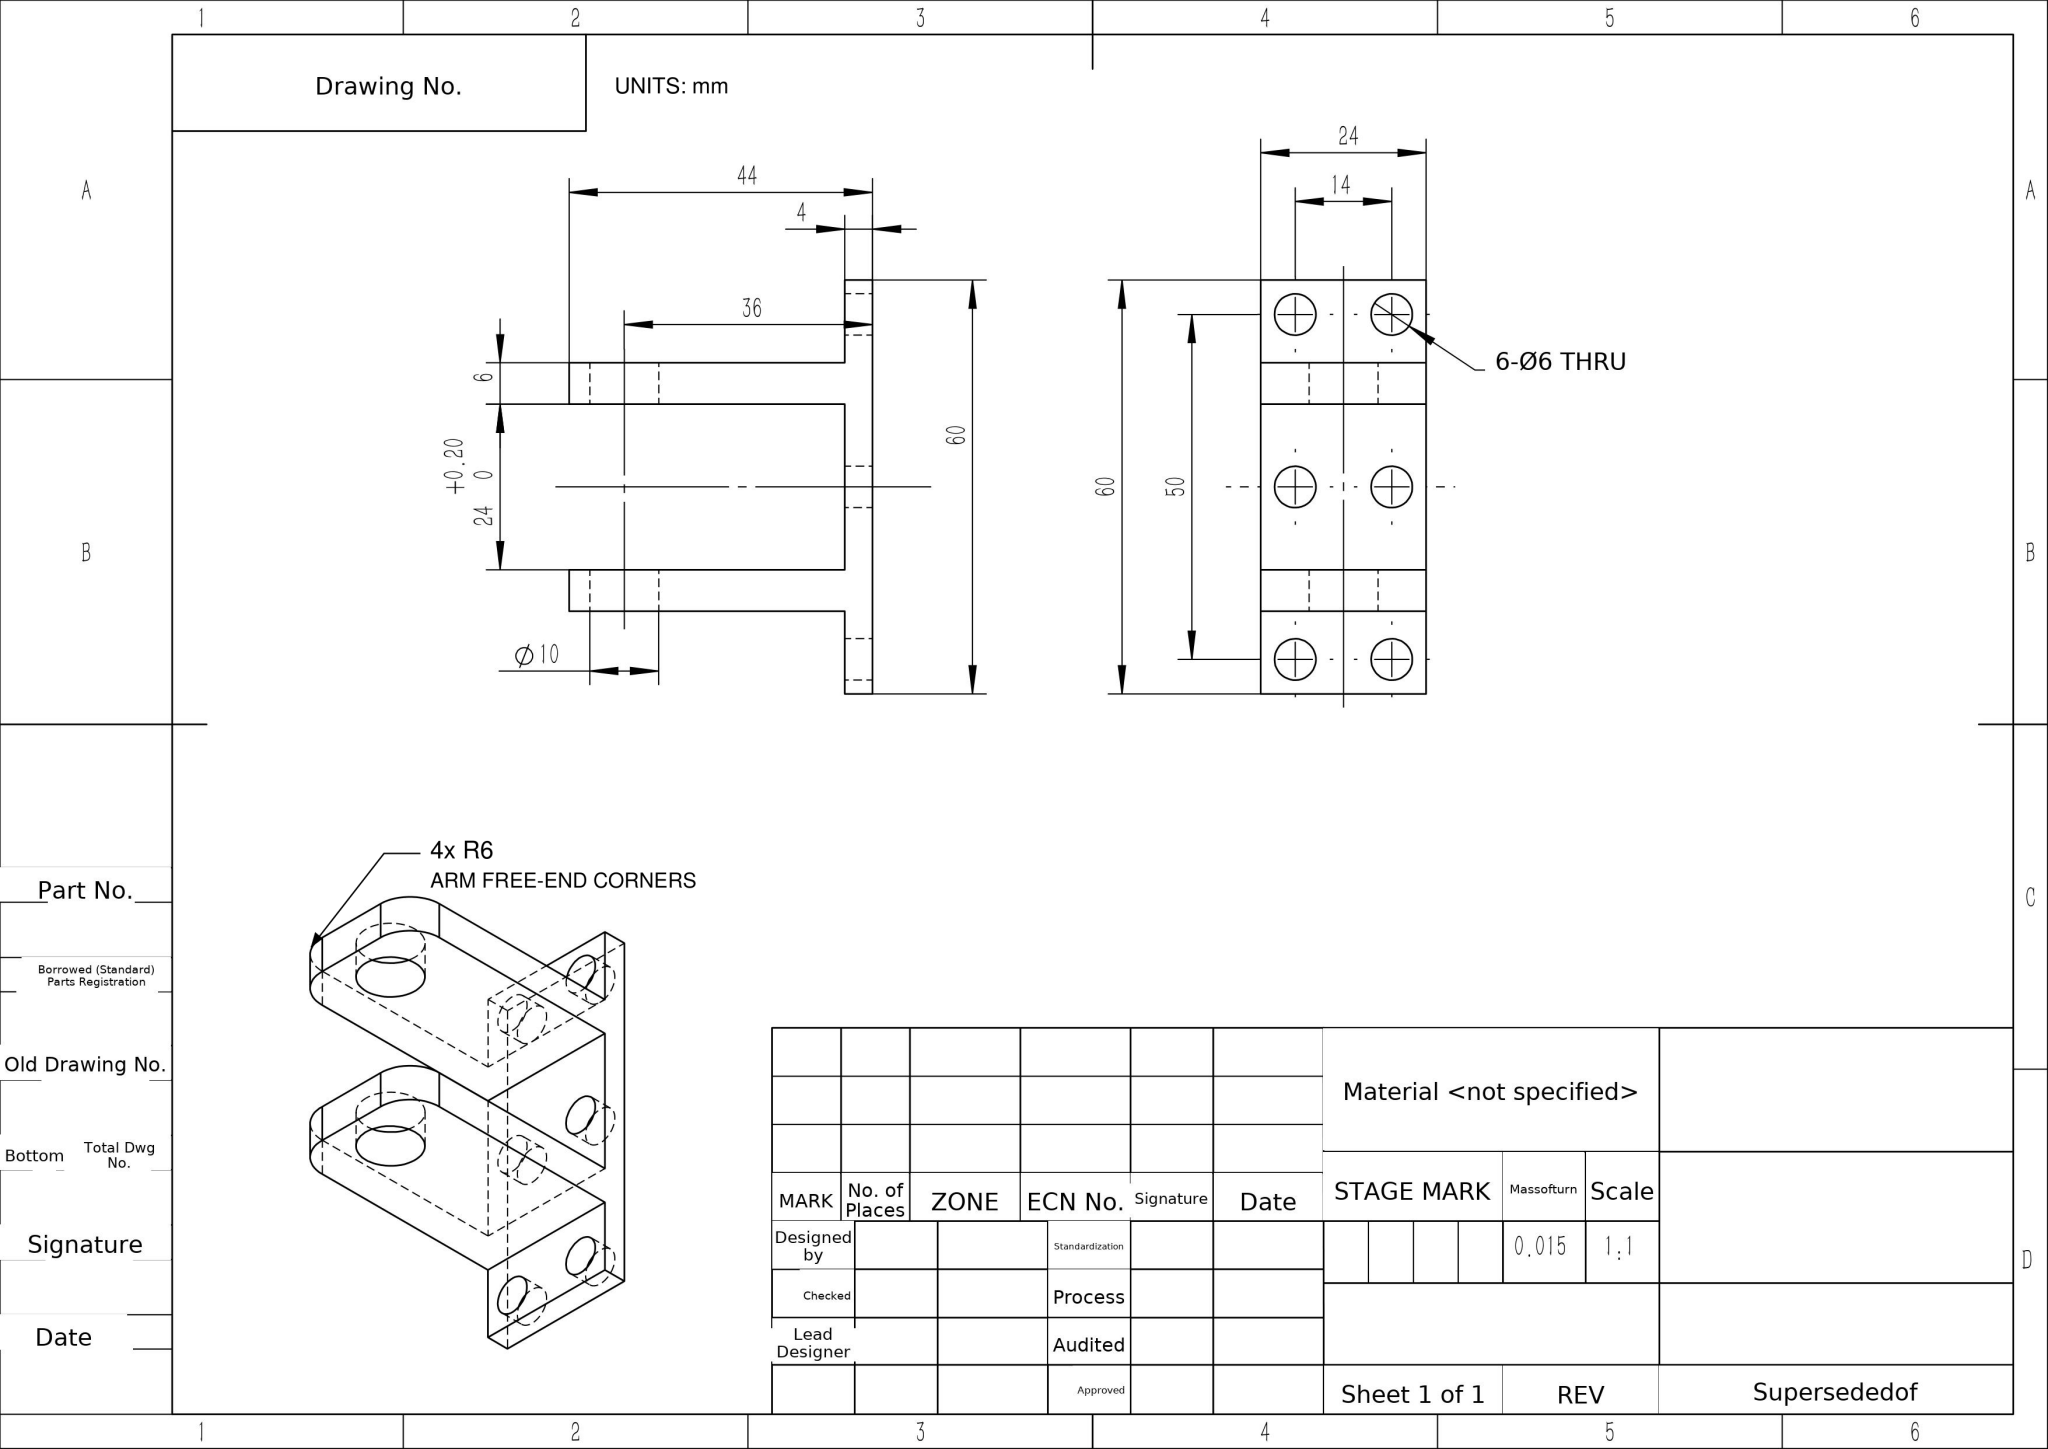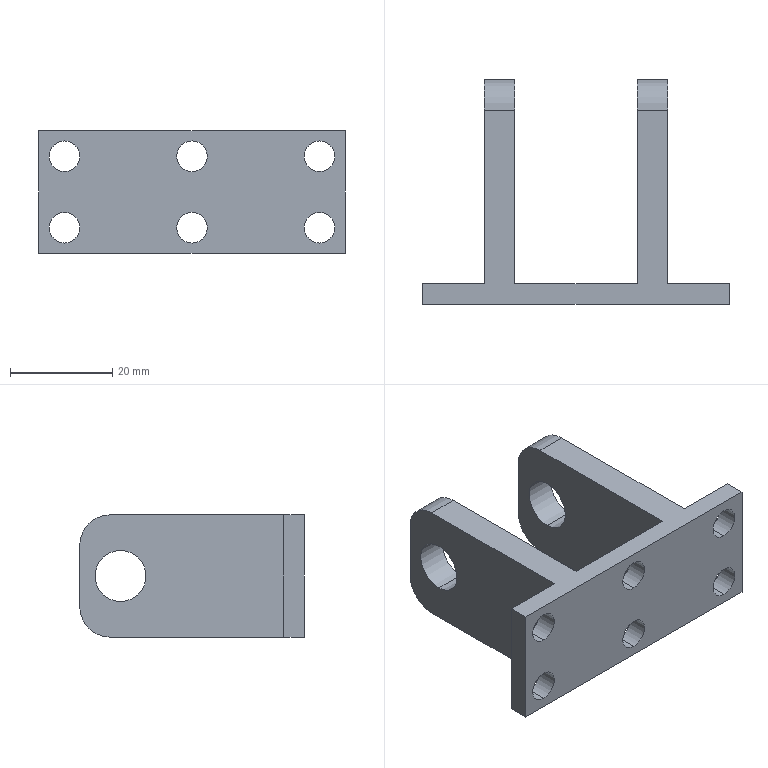Part | NX | mm | 1 solid | 34 faces | box 60 x 44 x 24 mm | volume 15474 mm3 | cylinder 20 | plane 14 | commonest cylinder face diameters 6 x12 10 x4 12 x4